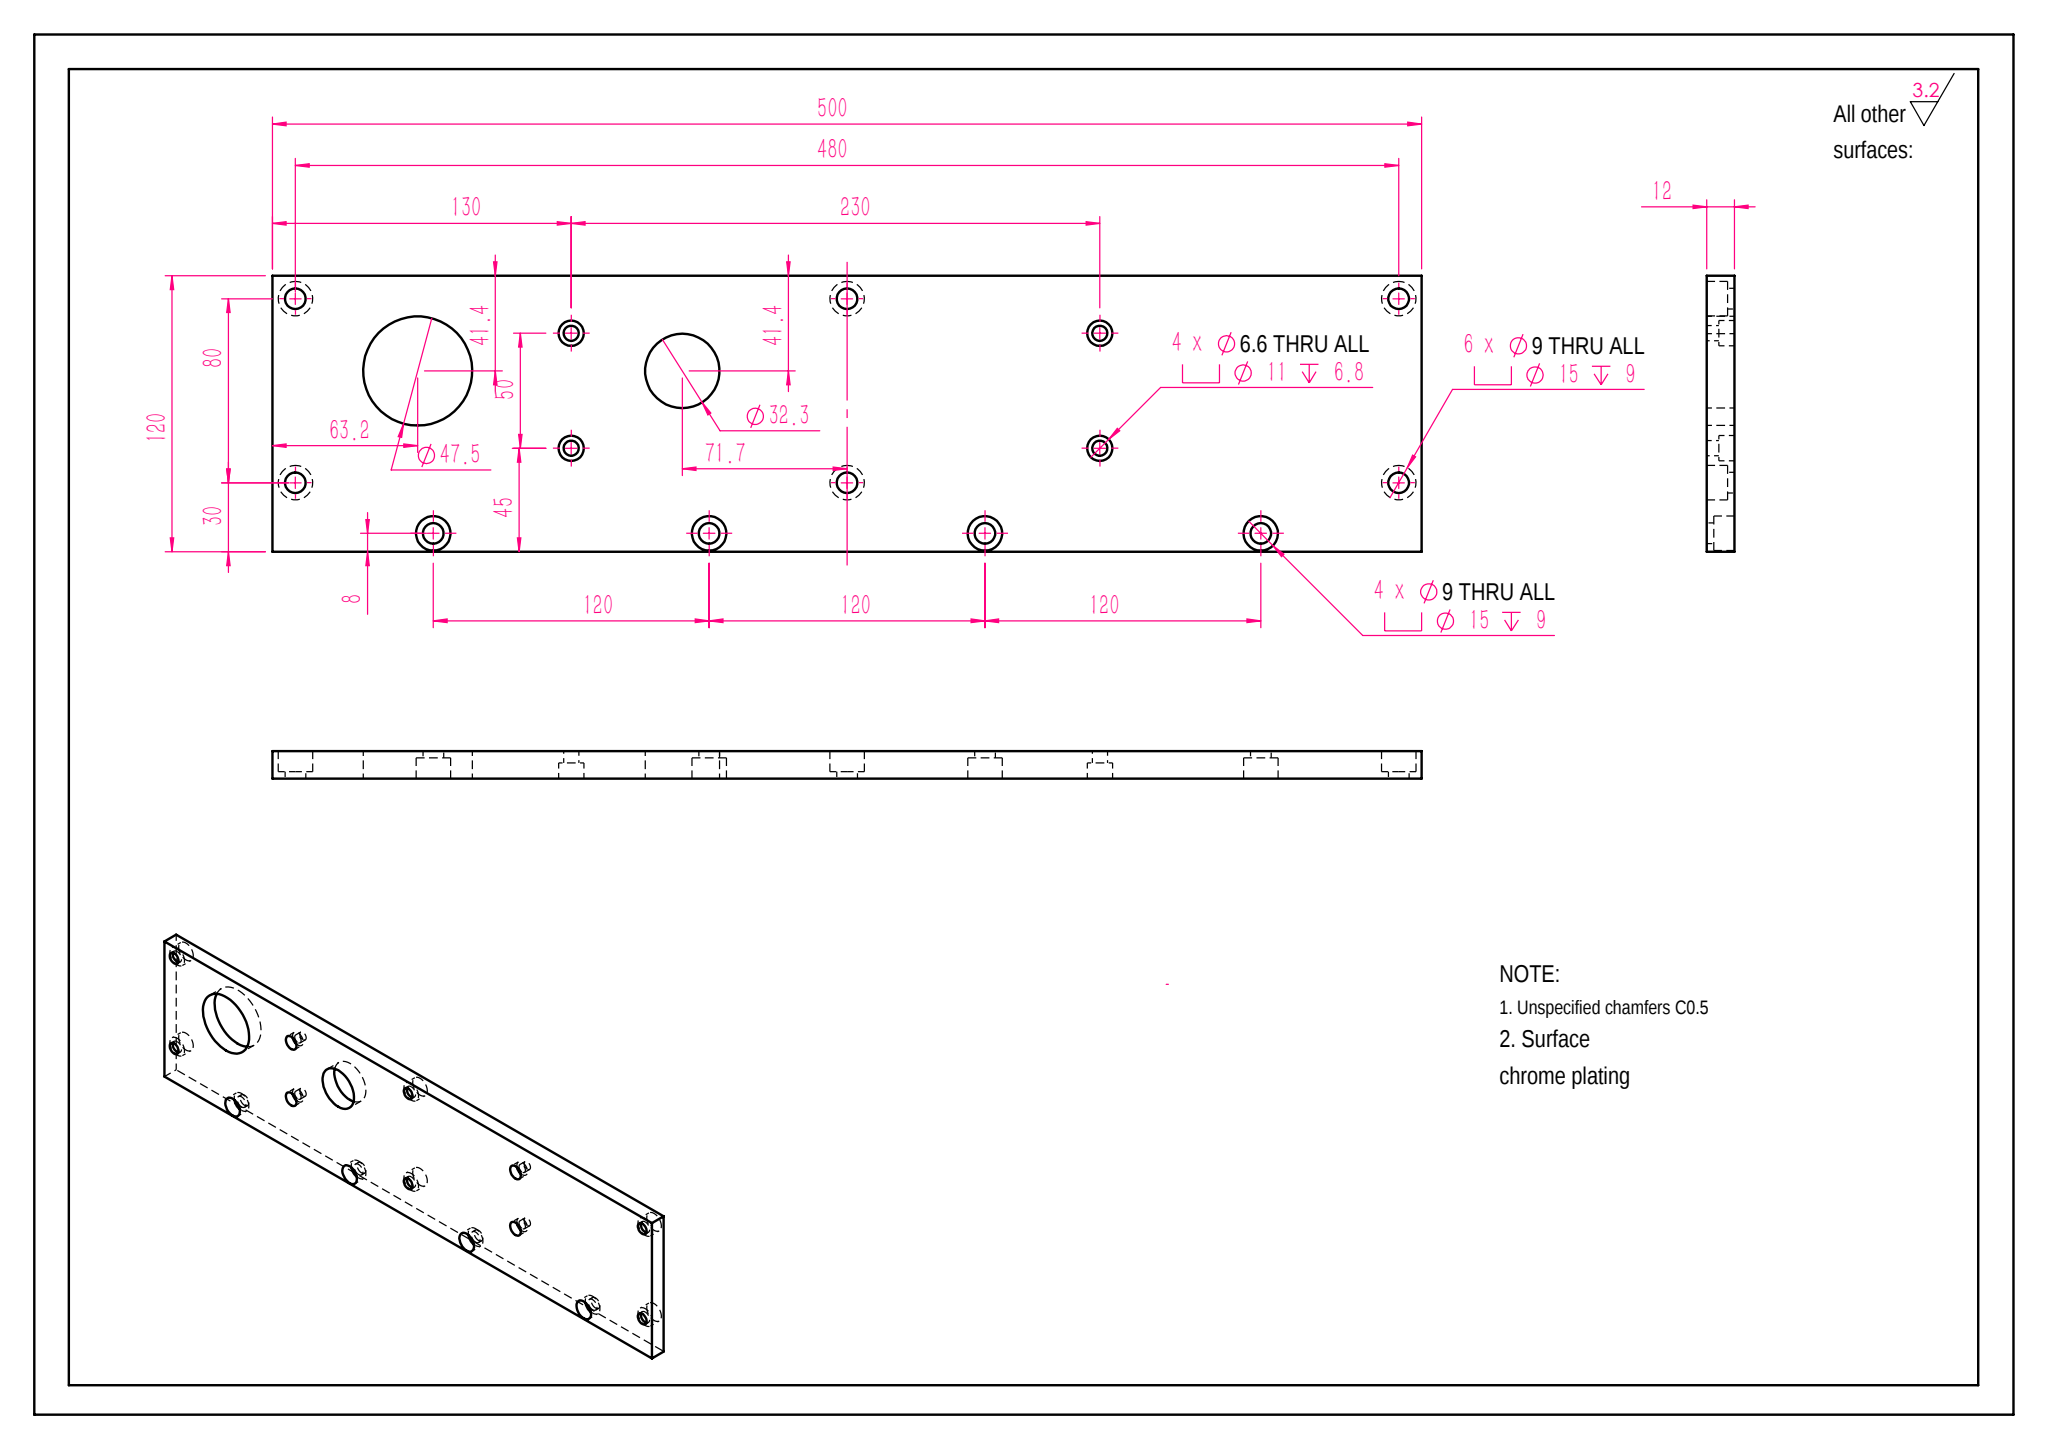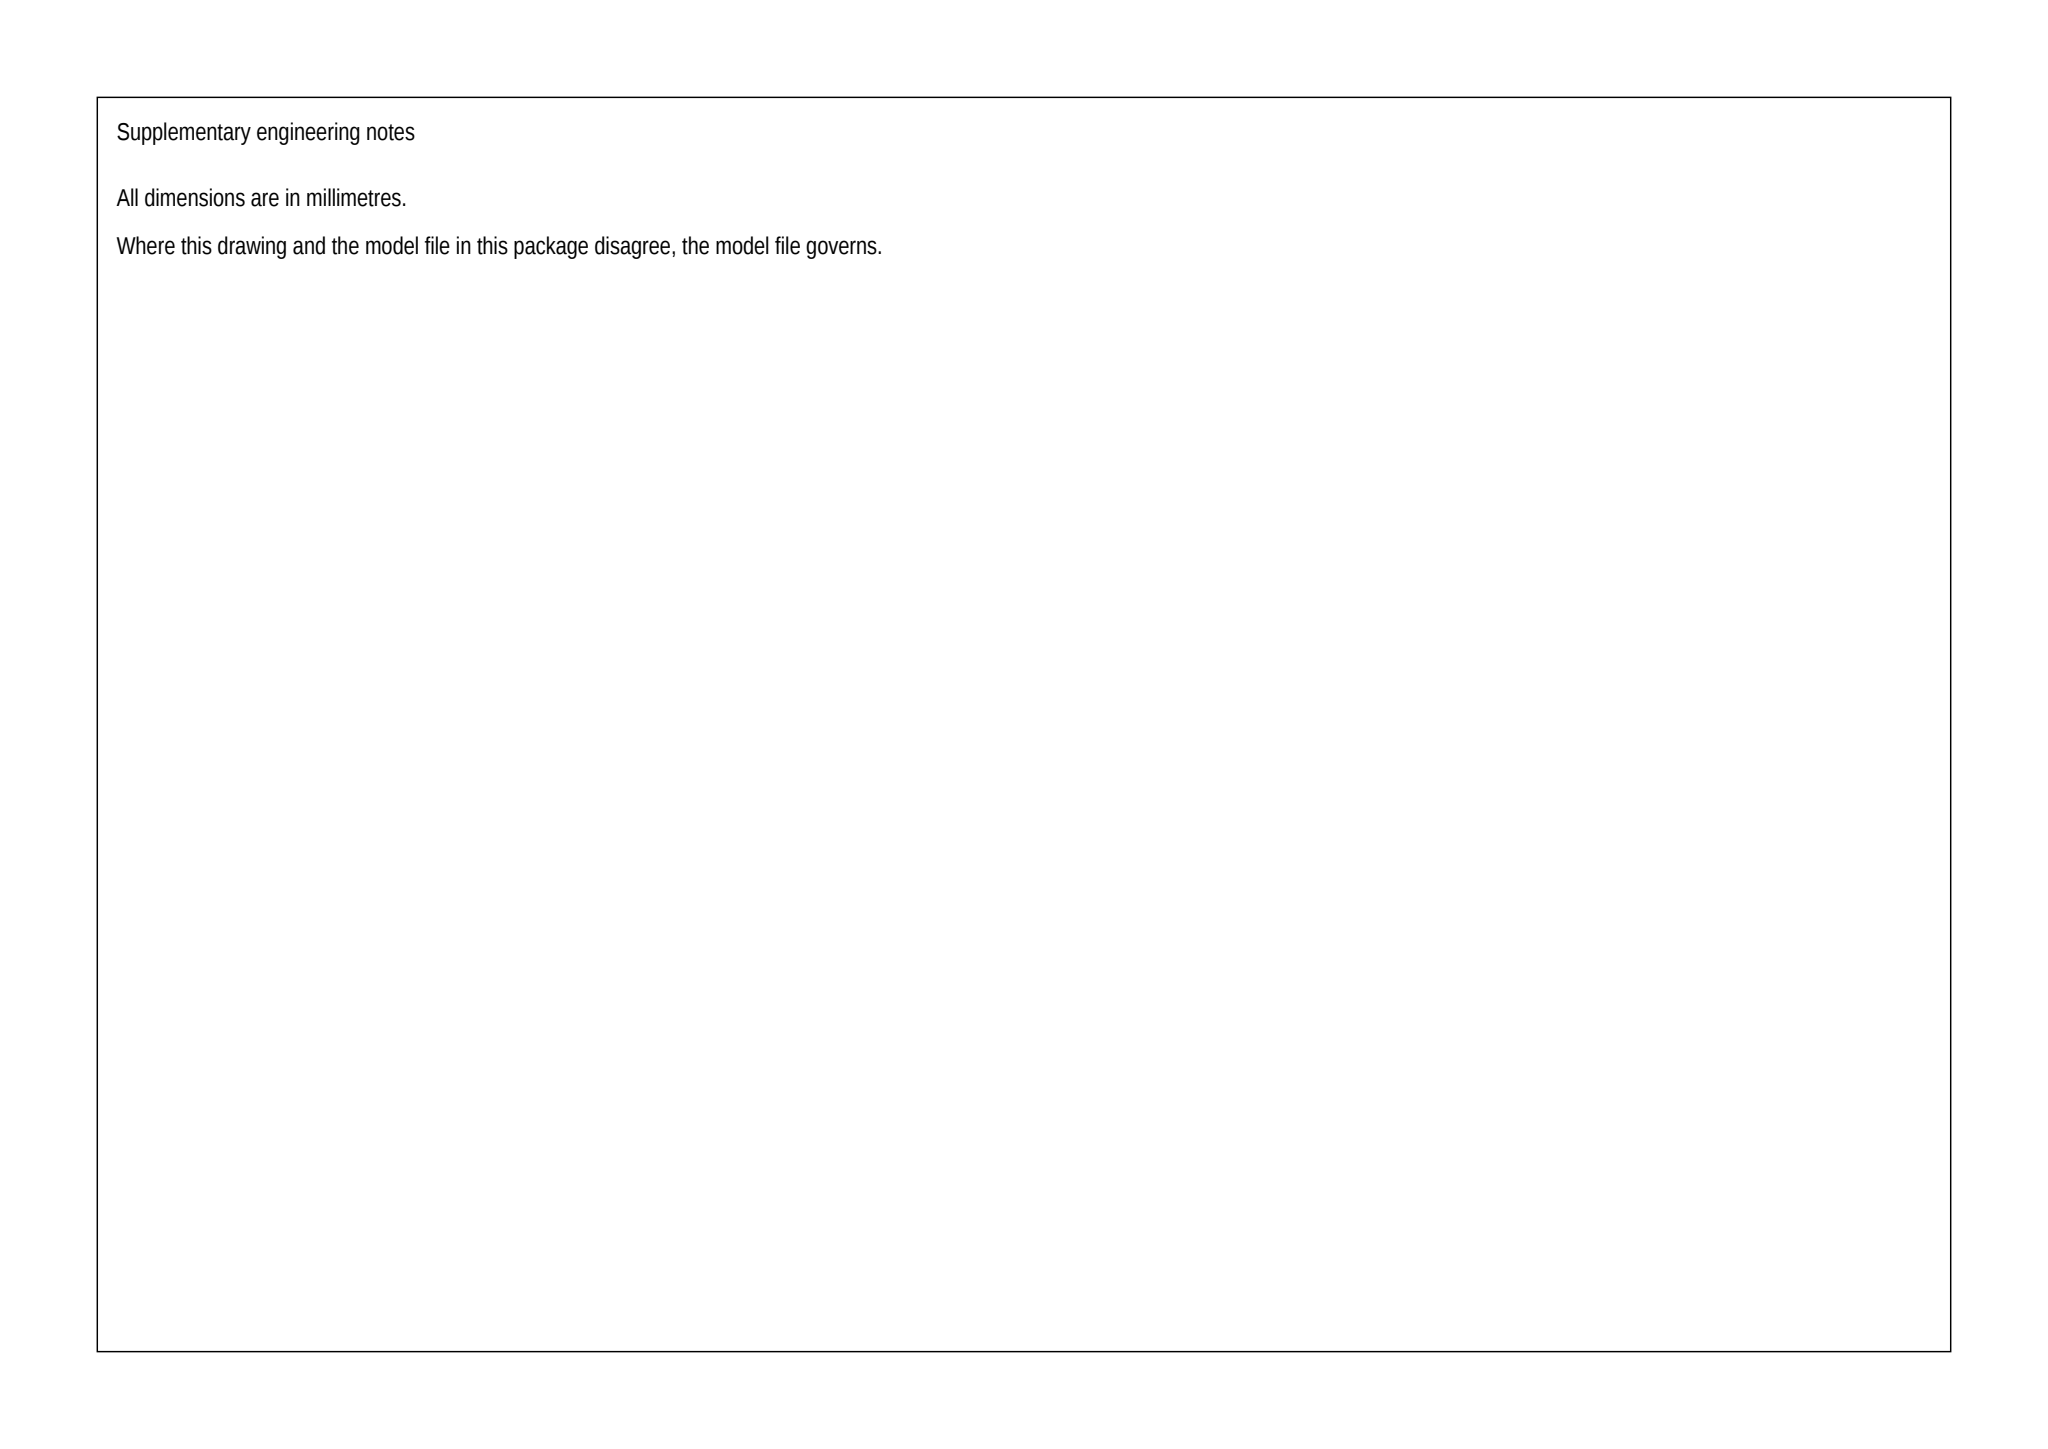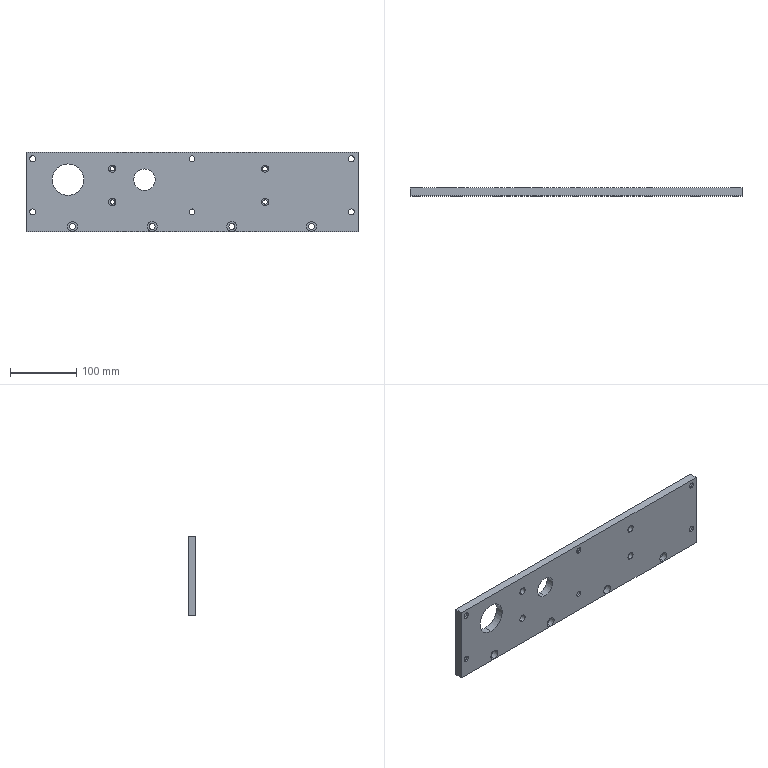Part | SolidWorks | mm | 1 solid | 80 faces | box 500 x 12 x 120 mm | volume 667825 mm3 | cylinder 60 | plane 20 | commonest cylinder face diameters 15 x20 9 x20 11 x8 6.6 x8 32.317 x2 47.453 x2
build123d program:
from build123d import *

# Parameters (mm, degrees)
SKETCH1_W                                            = 500
SKETCH1_H                                            = 120
BOSS_EXTRUDE1_DEPTH                                  = 12
HOLE_SIZE_ACCORDING_TO_HEXAGON_SOCKET_HE_D           = 9
HOLE_SIZE_ACCORDING_TO_HEXAGON_SOCKET_HE_CBORE_D     = 15
HOLE_SIZE_ACCORDING_TO_HEXAGON_SOCKET_HE_CBORE_DEPTH = 9
HOLE_SIZE_ACCORDING_TO_HEXAGON_SOCKE_2_D             = 9
HOLE_SIZE_ACCORDING_TO_HEXAGON_SOCKE_2_CBORE_D       = 15
HOLE_SIZE_ACCORDING_TO_HEXAGON_SOCKE_2_CBORE_DEPTH   = 9
HOLE_SIZE_ACCORDING_TO_HEXAGON_SOCKE_3_D             = 6.6
HOLE_SIZE_ACCORDING_TO_HEXAGON_SOCKE_3_CBORE_D       = 11
HOLE_SIZE_ACCORDING_TO_HEXAGON_SOCKE_3_CBORE_DEPTH   = 6.8
SKETCH10_R                                           = 16.158
SKETCH10_R_2                                         = 23.726
CUT_EXTRUDE1_DEPTH                                   = 80


with BuildPart() as part:
    # Sketch1 → Boss-Extrude1 (new body)
    with BuildSketch(Plane(origin=(0, 0, 0), x_dir=(1, 0, 0), z_dir=(0, 1, 0))):
        Rectangle(SKETCH1_W, SKETCH1_H)
    extrude(amount=BOSS_EXTRUDE1_DEPTH)

    # Hole Size according to Hexagon Socket He (through all)
    with Locations(Plane(origin=(0, 12, 0), x_dir=(1, 0, 0), z_dir=(0, 1, 0))):
        with Locations((-240, 30), (-240, -50), (0, 30), (0, -50), (240, 30), (240, -50)):
            CounterBoreHole(HOLE_SIZE_ACCORDING_TO_HEXAGON_SOCKET_HE_D / 2, HOLE_SIZE_ACCORDING_TO_HEXAGON_SOCKET_HE_CBORE_D / 2, HOLE_SIZE_ACCORDING_TO_HEXAGON_SOCKET_HE_CBORE_DEPTH)

    # Hole Size according to Hexagon Socke 2 (through all)
    with Locations(Plane(origin=(0, 0, 0), x_dir=(-1, 0, 0), z_dir=(0, -1, 0))):
        with Locations((180, 52), (60, 52), (-60, 52), (-180, 52)):
            CounterBoreHole(HOLE_SIZE_ACCORDING_TO_HEXAGON_SOCKE_2_D / 2, HOLE_SIZE_ACCORDING_TO_HEXAGON_SOCKE_2_CBORE_D / 2, HOLE_SIZE_ACCORDING_TO_HEXAGON_SOCKE_2_CBORE_DEPTH)

    # Hole Size according to Hexagon Socke 3 (through all)
    with Locations(Plane(origin=(0, 0, 0), x_dir=(-1, 0, 0), z_dir=(0, -1, 0))):
        with Locations((120, -35), (120, 15), (-110, -35), (-110, 15)):
            CounterBoreHole(HOLE_SIZE_ACCORDING_TO_HEXAGON_SOCKE_3_D / 2, HOLE_SIZE_ACCORDING_TO_HEXAGON_SOCKE_3_CBORE_D / 2, HOLE_SIZE_ACCORDING_TO_HEXAGON_SOCKE_3_CBORE_DEPTH)

    # Sketch10 → Cut-Extrude1 (cut)
    with BuildSketch(Plane(origin=(0, 0, 0), x_dir=(-1, 0, 0), z_dir=(0, -1, 0))):
        with Locations(Location((71.663, -18.621, 0), (0, 0, 90))):
            Circle(SKETCH10_R)
        with Locations(Location((186.775, -18.621, 0), (0, 0, 90))):
            Circle(SKETCH10_R_2)
    extrude(amount=-CUT_EXTRUDE1_DEPTH, mode=Mode.SUBTRACT)


solid = part.part